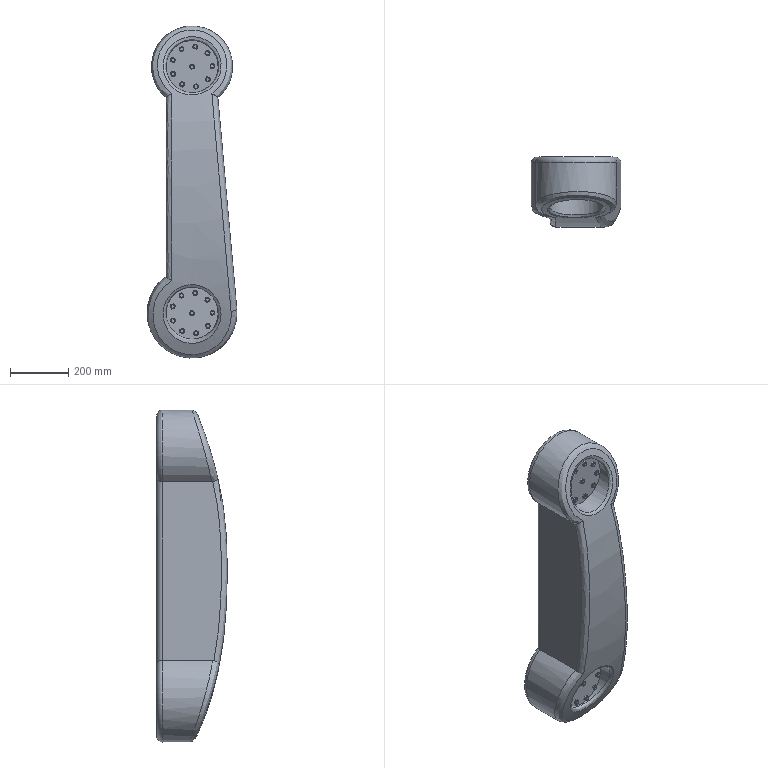Component | NX | 3_SHOULDER | 23 solids | 208 faces | volume 50663172 mm3 | plane 169 | other 21 | cylinder 10 | spline 6 | torus 2 | commonest cylinder face diameters 180 x4 20 x2 40 x2 280 x1 310 x1